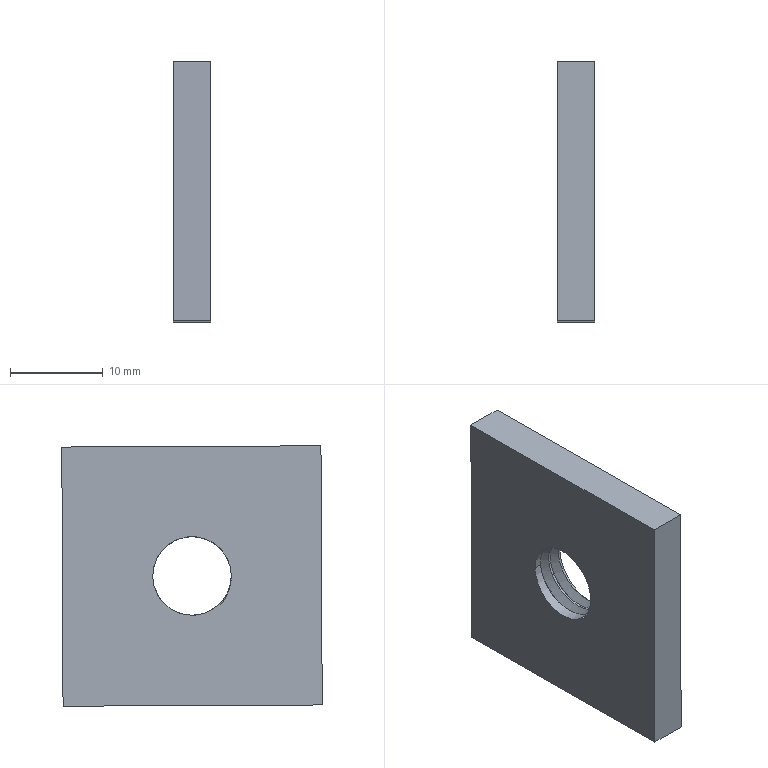Component | SolidWorks | GroundingDeviceAssembly-1_GroundingCopperBlock-1 | 1 solid | 16 faces | box 4 x 28.13 x 28.13 mm | volume 2875 mm3 | cylinder 7 | plane 7 | spline 2 | commonest cylinder face diameters 8.5 x7
STEP:
#1=COLOUR_RGB('',0.7922,0.8196,0.9333);
#2=FILL_AREA_STYLE_COLOUR('',#1);
#3=FILL_AREA_STYLE('',(#2));
#4=SURFACE_STYLE_FILL_AREA(#3);
#5=SURFACE_SIDE_STYLE('',(#4));
#6=SURFACE_STYLE_USAGE(.BOTH.,#5);
#7=PRESENTATION_STYLE_ASSIGNMENT((#6));
#8=CARTESIAN_POINT('',(29.241,-7.002,9.527));
#9=VERTEX_POINT('',#8);
#10=CARTESIAN_POINT('',(29.212,-7.337,9.528));
#11=VERTEX_POINT('',#10);
#12=CARTESIAN_POINT('',(29.241,-7.002,9.527));
#13=CARTESIAN_POINT('',(29.238,-7.002,9.596));
#14=CARTESIAN_POINT('',(29.234,-7.051,9.645));
#15=CARTESIAN_POINT('',(29.23,-7.099,9.695));
#16=CARTESIAN_POINT('',(29.227,-7.169,9.695));
#17=CARTESIAN_POINT('',(29.223,-7.238,9.695));
#18=CARTESIAN_POINT('',(29.219,-7.287,9.646));
#19=CARTESIAN_POINT('',(29.216,-7.336,9.598));
#20=CARTESIAN_POINT('',(29.212,-7.337,9.528));
#21=(BOUNDED_CURVE()B_SPLINE_CURVE(2,(#12,#13,#14,#15,#16,#17,#18,#19,#20),.UNSPECIFIED.,.F.,.F.)B_SPLINE_CURVE_WITH_KNOTS((3,2,2,2,3),(0.4583,0.5,0.5417,0.5833,0.625),.UNSPECIFIED.)CURVE()GEOMETRIC_REPRESENTATION_ITEM()RATIONAL_B_SPLINE_CURVE((1.,0.9239,1.,0.9239,1.,0.9239,1.,0.9239,1.))REPRESENTATION_ITEM(''));
#22=EDGE_CURVE('',#9,#11,#21,.T.);
#23=ORIENTED_EDGE('',*,*,#22,.F.);
#24=CARTESIAN_POINT('',(29.251,-7.002,9.527));
#25=VERTEX_POINT('',#24);
#26=CARTESIAN_POINT('',(29.061,-7.002,9.527));
#27=DIRECTION('',(1.,0.,-0.));
#28=VECTOR('',#27,39.37);
#29=LINE('',#26,#28);
#30=EDGE_CURVE('',#9,#25,#29,.T.);
#31=ORIENTED_EDGE('',*,*,#30,.T.);
#32=CARTESIAN_POINT('',(29.222,-7.337,9.528));
#33=VERTEX_POINT('',#32);
#34=CARTESIAN_POINT('',(29.222,-7.337,9.528));
#35=CARTESIAN_POINT('',(29.225,-7.336,9.598));
#36=CARTESIAN_POINT('',(29.229,-7.287,9.646));
#37=CARTESIAN_POINT('',(29.233,-7.238,9.695));
#38=CARTESIAN_POINT('',(29.236,-7.169,9.695));
#39=CARTESIAN_POINT('',(29.24,-7.099,9.695));
#40=CARTESIAN_POINT('',(29.244,-7.051,9.645));
#41=CARTESIAN_POINT('',(29.247,-7.002,9.596));
#42=CARTESIAN_POINT('',(29.251,-7.002,9.527));
#43=(BOUNDED_CURVE()B_SPLINE_CURVE(2,(#34,#35,#36,#37,#38,#39,#40,#41,#42),.UNSPECIFIED.,.F.,.F.)B_SPLINE_CURVE_WITH_KNOTS((3,2,2,2,3),(0.7083,0.75,0.7917,0.8333,0.875),.UNSPECIFIED.)CURVE()GEOMETRIC_REPRESENTATION_ITEM()RATIONAL_B_SPLINE_CURVE((1.,0.9239,1.,0.9239,1.,0.9239,1.,0.9239,1.))REPRESENTATION_ITEM(''));
#44=EDGE_CURVE('',#33,#25,#43,.T.);
#45=ORIENTED_EDGE('',*,*,#44,.F.);
#46=CARTESIAN_POINT('',(29.061,-7.337,9.528));
#47=DIRECTION('',(1.,0.,-0.));
#48=VECTOR('',#47,39.37);
#49=LINE('',#46,#48);
#50=EDGE_CURVE('',#11,#33,#49,.T.);
#51=ORIENTED_EDGE('',*,*,#50,.F.);
#52=EDGE_LOOP('',(#23,#31,#45,#51));
#53=FACE_OUTER_BOUND('',#52,.T.);
#54=CARTESIAN_POINT('',(29.061,-7.169,9.528));
#55=DIRECTION('',(1.,0.,-0.));
#56=DIRECTION('',(0.,-1.,0.004786));
#57=AXIS2_PLACEMENT_3D('',#54,#55,#56);
#58=CYLINDRICAL_SURFACE('',#57,0.1673);
#59=ADVANCED_FACE('',(#53),#58,.F.);
#60=CARTESIAN_POINT('',(29.1,-7.002,9.527));
#61=VERTEX_POINT('',#60);
#62=CARTESIAN_POINT('',(29.1,-7.337,9.528));
#63=VERTEX_POINT('',#62);
#64=CARTESIAN_POINT('',(29.1,-7.169,9.528));
#65=DIRECTION('',(1.,0.,-0.));
#66=DIRECTION('',(0.,-1.,0.004786));
#67=AXIS2_PLACEMENT_3D('',#64,#65,#66);
#68=CIRCLE('',#67,0.1673);
#69=EDGE_CURVE('',#61,#63,#68,.T.);
#70=ORIENTED_EDGE('',*,*,#69,.F.);
#71=CARTESIAN_POINT('',(29.133,-7.002,9.527));
#72=VERTEX_POINT('',#71);
#73=CARTESIAN_POINT('',(29.061,-7.002,9.527));
#74=DIRECTION('',(1.,0.,-0.));
#75=VECTOR('',#74,39.37);
#76=LINE('',#73,#75);
#77=EDGE_CURVE('',#61,#72,#76,.T.);
#78=ORIENTED_EDGE('',*,*,#77,.T.);
#79=CARTESIAN_POINT('',(29.103,-7.337,9.528));
#80=VERTEX_POINT('',#79);
#81=CARTESIAN_POINT('',(29.103,-7.337,9.528));
#82=CARTESIAN_POINT('',(29.107,-7.336,9.598));
#83=CARTESIAN_POINT('',(29.111,-7.287,9.646));
#84=CARTESIAN_POINT('',(29.115,-7.238,9.695));
#85=CARTESIAN_POINT('',(29.118,-7.169,9.695));
#86=CARTESIAN_POINT('',(29.122,-7.099,9.695));
#87=CARTESIAN_POINT('',(29.126,-7.051,9.645));
#88=CARTESIAN_POINT('',(29.129,-7.002,9.596));
#89=CARTESIAN_POINT('',(29.133,-7.002,9.527));
#90=(BOUNDED_CURVE()B_SPLINE_CURVE(2,(#81,#82,#83,#84,#85,#86,#87,#88,#89),.UNSPECIFIED.,.F.,.F.)B_SPLINE_CURVE_WITH_KNOTS((3,2,2,2,3),(0.04167,0.08333,0.125,0.1667,0.2083),.UNSPECIFIED.)CURVE()GEOMETRIC_REPRESENTATION_ITEM()RATIONAL_B_SPLINE_CURVE((1.,0.9239,1.,0.9239,1.,0.9239,1.,0.9239,1.))REPRESENTATION_ITEM(''));
#91=EDGE_CURVE('',#80,#72,#90,.T.);
#92=ORIENTED_EDGE('',*,*,#91,.F.);
#93=CARTESIAN_POINT('',(29.061,-7.337,9.528));
#94=DIRECTION('',(1.,0.,-0.));
#95=VECTOR('',#94,39.37);
#96=LINE('',#93,#95);
#97=EDGE_CURVE('',#63,#80,#96,.T.);
#98=ORIENTED_EDGE('',*,*,#97,.F.);
#99=EDGE_LOOP('',(#70,#78,#92,#98));
#100=FACE_OUTER_BOUND('',#99,.T.);
#101=CARTESIAN_POINT('',(29.061,-7.169,9.528));
#102=DIRECTION('',(1.,0.,-0.));
#103=DIRECTION('',(0.,-1.,0.004786));
#104=AXIS2_PLACEMENT_3D('',#101,#102,#103);
#105=CYLINDRICAL_SURFACE('',#104,0.1673);
#106=ADVANCED_FACE('',(#100),#105,.F.);
#107=CARTESIAN_POINT('',(29.182,-7.002,9.527));
#108=VERTEX_POINT('',#107);
#109=CARTESIAN_POINT('',(29.153,-7.337,9.528));
#110=VERTEX_POINT('',#109);
#111=CARTESIAN_POINT('',(29.182,-7.002,9.527));
#112=CARTESIAN_POINT('',(29.179,-7.002,9.596));
#113=CARTESIAN_POINT('',(29.175,-7.051,9.645));
#114=CARTESIAN_POINT('',(29.171,-7.099,9.695));
#115=CARTESIAN_POINT('',(29.168,-7.169,9.695));
#116=CARTESIAN_POINT('',(29.164,-7.238,9.695));
#117=CARTESIAN_POINT('',(29.16,-7.287,9.646));
#118=CARTESIAN_POINT('',(29.157,-7.336,9.598));
#119=CARTESIAN_POINT('',(29.153,-7.337,9.528));
#120=(BOUNDED_CURVE()B_SPLINE_CURVE(2,(#111,#112,#113,#114,#115,#116,#117,#118,#119),.UNSPECIFIED.,.F.,.F.)B_SPLINE_CURVE_WITH_KNOTS((3,2,2,2,3),(0.7917,0.8333,0.875,0.9167,0.9583),.UNSPECIFIED.)CURVE()GEOMETRIC_REPRESENTATION_ITEM()RATIONAL_B_SPLINE_CURVE((1.,0.9239,1.,0.9239,1.,0.9239,1.,0.9239,1.))REPRESENTATION_ITEM(''));
#121=EDGE_CURVE('',#108,#110,#120,.T.);
#122=ORIENTED_EDGE('',*,*,#121,.F.);
#123=CARTESIAN_POINT('',(29.192,-7.002,9.527));
#124=VERTEX_POINT('',#123);
#125=CARTESIAN_POINT('',(29.061,-7.002,9.527));
#126=DIRECTION('',(1.,0.,-0.));
#127=VECTOR('',#126,39.37);
#128=LINE('',#125,#127);
#129=EDGE_CURVE('',#108,#124,#128,.T.);
#130=ORIENTED_EDGE('',*,*,#129,.T.);
#131=CARTESIAN_POINT('',(29.163,-7.337,9.528));
#132=VERTEX_POINT('',#131);
#133=CARTESIAN_POINT('',(29.163,-7.337,9.528));
#134=CARTESIAN_POINT('',(29.166,-7.336,9.598));
#135=CARTESIAN_POINT('',(29.17,-7.287,9.646));
#136=CARTESIAN_POINT('',(29.174,-7.238,9.695));
#137=CARTESIAN_POINT('',(29.177,-7.169,9.695));
#138=CARTESIAN_POINT('',(29.181,-7.099,9.695));
#139=CARTESIAN_POINT('',(29.185,-7.051,9.645));
#140=CARTESIAN_POINT('',(29.188,-7.002,9.596));
#141=CARTESIAN_POINT('',(29.192,-7.002,9.527));
#142=(BOUNDED_CURVE()B_SPLINE_CURVE(2,(#133,#134,#135,#136,#137,#138,#139,#140,#141),.UNSPECIFIED.,.F.,.F.)B_SPLINE_CURVE_WITH_KNOTS((3,2,2,2,3),(0.375,0.4167,0.4583,0.5,0.5417),.UNSPECIFIED.)CURVE()GEOMETRIC_REPRESENTATION_ITEM()RATIONAL_B_SPLINE_CURVE((1.,0.9239,1.,0.9239,1.,0.9239,1.,0.9239,1.))REPRESENTATION_ITEM(''));
#143=EDGE_CURVE('',#132,#124,#142,.T.);
#144=ORIENTED_EDGE('',*,*,#143,.F.);
#145=CARTESIAN_POINT('',(29.061,-7.337,9.528));
#146=DIRECTION('',(1.,0.,-0.));
#147=VECTOR('',#146,39.37);
#148=LINE('',#145,#147);
#149=EDGE_CURVE('',#110,#132,#148,.T.);
#150=ORIENTED_EDGE('',*,*,#149,.F.);
#151=EDGE_LOOP('',(#122,#130,#144,#150));
#152=FACE_OUTER_BOUND('',#151,.T.);
#153=CARTESIAN_POINT('',(29.061,-7.169,9.528));
#154=DIRECTION('',(1.,0.,-0.));
#155=DIRECTION('',(0.,-1.,0.004786));
#156=AXIS2_PLACEMENT_3D('',#153,#154,#155);
#157=CYLINDRICAL_SURFACE('',#156,0.1673);
#158=ADVANCED_FACE('',(#152),#157,.F.);
#159=CARTESIAN_POINT('',(29.1,-7.329,9.476));
#160=VERTEX_POINT('',#159);
#161=CARTESIAN_POINT('',(29.1,-7.169,9.528));
#162=DIRECTION('',(1.,0.,-0.));
#163=DIRECTION('',(0.,-1.,0.004786));
#164=AXIS2_PLACEMENT_3D('',#161,#162,#163);
#165=CIRCLE('',#164,0.1673);
#166=EDGE_CURVE('',#63,#160,#165,.T.);
#167=ORIENTED_EDGE('',*,*,#166,.F.);
#168=ORIENTED_EDGE('',*,*,#97,.T.);
#169=CARTESIAN_POINT('',(29.1,-7.329,9.476));
#170=CARTESIAN_POINT('',(29.102,-7.337,9.501));
#171=CARTESIAN_POINT('',(29.103,-7.337,9.528));
#172=(BOUNDED_CURVE()B_SPLINE_CURVE(2,(#169,#170,#171),.UNSPECIFIED.,.F.,.F.)B_SPLINE_CURVE_WITH_KNOTS((3,3),(0.02463,0.04167),.UNSPECIFIED.)CURVE()GEOMETRIC_REPRESENTATION_ITEM()RATIONAL_B_SPLINE_CURVE((0.9632,0.9689,1.))REPRESENTATION_ITEM(''));
#173=EDGE_CURVE('',#160,#80,#172,.T.);
#174=ORIENTED_EDGE('',*,*,#173,.F.);
#175=EDGE_LOOP('',(#167,#168,#174));
#176=FACE_OUTER_BOUND('',#175,.T.);
#177=CARTESIAN_POINT('',(29.061,-7.169,9.528));
#178=DIRECTION('',(1.,0.,-0.));
#179=DIRECTION('',(0.,-1.,0.004786));
#180=AXIS2_PLACEMENT_3D('',#177,#178,#179);
#181=CYLINDRICAL_SURFACE('',#180,0.1673);
#182=ADVANCED_FACE('',(#176),#181,.F.);
#183=ORIENTED_EDGE('',*,*,#77,.F.);
#184=CARTESIAN_POINT('',(29.1,-7.288,9.41));
#185=VERTEX_POINT('',#184);
#186=CARTESIAN_POINT('',(29.1,-7.169,9.528));
#187=DIRECTION('',(1.,0.,-0.));
#188=DIRECTION('',(0.,-1.,0.004786));
#189=AXIS2_PLACEMENT_3D('',#186,#187,#188);
#190=CIRCLE('',#189,0.1673);
#191=EDGE_CURVE('',#185,#61,#190,.T.);
#192=ORIENTED_EDGE('',*,*,#191,.F.);
#193=CARTESIAN_POINT('',(29.145,-7.288,9.41));
#194=VERTEX_POINT('',#193);
#195=CARTESIAN_POINT('',(29.061,-7.288,9.41));
#196=DIRECTION('',(1.,0.,-0.));
#197=VECTOR('',#196,39.37);
#198=LINE('',#195,#197);
#199=EDGE_CURVE('',#185,#194,#198,.T.);
#200=ORIENTED_EDGE('',*,*,#199,.T.);
#201=CARTESIAN_POINT('',(29.153,-7.337,9.528));
#202=CARTESIAN_POINT('',(29.149,-7.337,9.459));
#203=CARTESIAN_POINT('',(29.145,-7.288,9.41));
#204=(BOUNDED_CURVE()B_SPLINE_CURVE(2,(#201,#202,#203),.UNSPECIFIED.,.F.,.F.)B_SPLINE_CURVE_WITH_KNOTS((3,3),(0.9583,1.),.UNSPECIFIED.)CURVE()GEOMETRIC_REPRESENTATION_ITEM()RATIONAL_B_SPLINE_CURVE((1.,0.9239,1.))REPRESENTATION_ITEM(''));
#205=EDGE_CURVE('',#110,#194,#204,.T.);
#206=ORIENTED_EDGE('',*,*,#205,.F.);
#207=ORIENTED_EDGE('',*,*,#149,.T.);
#208=CARTESIAN_POINT('',(29.133,-7.002,9.527));
#209=CARTESIAN_POINT('',(29.137,-7.002,9.457));
#210=CARTESIAN_POINT('',(29.14,-7.052,9.409));
#211=CARTESIAN_POINT('',(29.144,-7.101,9.36));
#212=CARTESIAN_POINT('',(29.148,-7.17,9.36));
#213=CARTESIAN_POINT('',(29.151,-7.24,9.361));
#214=CARTESIAN_POINT('',(29.155,-7.288,9.41));
#215=CARTESIAN_POINT('',(29.159,-7.337,9.459));
#216=CARTESIAN_POINT('',(29.163,-7.337,9.528));
#217=(BOUNDED_CURVE()B_SPLINE_CURVE(2,(#208,#209,#210,#211,#212,#213,#214,#215,#216),.UNSPECIFIED.,.F.,.F.)B_SPLINE_CURVE_WITH_KNOTS((3,2,2,2,3),(0.2083,0.25,0.2917,0.3333,0.375),.UNSPECIFIED.)CURVE()GEOMETRIC_REPRESENTATION_ITEM()RATIONAL_B_SPLINE_CURVE((1.,0.9239,1.,0.9239,1.,0.9239,1.,0.9239,1.))REPRESENTATION_ITEM(''));
#218=EDGE_CURVE('',#72,#132,#217,.T.);
#219=ORIENTED_EDGE('',*,*,#218,.F.);
#220=EDGE_LOOP('',(#183,#192,#200,#206,#207,#219));
#221=FACE_OUTER_BOUND('',#220,.T.);
#222=CARTESIAN_POINT('',(29.061,-7.169,9.528));
#223=DIRECTION('',(1.,0.,-0.));
#224=DIRECTION('',(0.,-1.,0.004786));
#225=AXIS2_PLACEMENT_3D('',#222,#223,#224);
#226=CYLINDRICAL_SURFACE('',#225,0.1673);
#227=ADVANCED_FACE('',(#221),#226,.F.);
#228=ORIENTED_EDGE('',*,*,#129,.F.);
#229=CARTESIAN_POINT('',(29.212,-7.337,9.528));
#230=CARTESIAN_POINT('',(29.208,-7.337,9.459));
#231=CARTESIAN_POINT('',(29.205,-7.288,9.41));
#232=CARTESIAN_POINT('',(29.201,-7.24,9.361));
#233=CARTESIAN_POINT('',(29.197,-7.17,9.36));
#234=CARTESIAN_POINT('',(29.193,-7.101,9.36));
#235=CARTESIAN_POINT('',(29.19,-7.052,9.409));
#236=CARTESIAN_POINT('',(29.186,-7.002,9.457));
#237=CARTESIAN_POINT('',(29.182,-7.002,9.527));
#238=(BOUNDED_CURVE()B_SPLINE_CURVE(2,(#229,#230,#231,#232,#233,#234,#235,#236,#237),.UNSPECIFIED.,.F.,.F.)B_SPLINE_CURVE_WITH_KNOTS((3,2,2,2,3),(0.625,0.6667,0.7083,0.75,0.7917),.UNSPECIFIED.)CURVE()GEOMETRIC_REPRESENTATION_ITEM()RATIONAL_B_SPLINE_CURVE((1.,0.9239,1.,0.9239,1.,0.9239,1.,0.9239,1.))REPRESENTATION_ITEM(''));
#239=EDGE_CURVE('',#11,#108,#238,.T.);
#240=ORIENTED_EDGE('',*,*,#239,.F.);
#241=ORIENTED_EDGE('',*,*,#50,.T.);
#242=CARTESIAN_POINT('',(29.192,-7.002,9.527));
#243=CARTESIAN_POINT('',(29.196,-7.002,9.457));
#244=CARTESIAN_POINT('',(29.199,-7.052,9.409));
#245=CARTESIAN_POINT('',(29.203,-7.101,9.36));
#246=CARTESIAN_POINT('',(29.207,-7.17,9.36));
#247=CARTESIAN_POINT('',(29.211,-7.24,9.361));
#248=CARTESIAN_POINT('',(29.214,-7.288,9.41));
#249=CARTESIAN_POINT('',(29.218,-7.337,9.459));
#250=CARTESIAN_POINT('',(29.222,-7.337,9.528));
#251=(BOUNDED_CURVE()B_SPLINE_CURVE(2,(#242,#243,#244,#245,#246,#247,#248,#249,#250),.UNSPECIFIED.,.F.,.F.)B_SPLINE_CURVE_WITH_KNOTS((3,2,2,2,3),(0.5417,0.5833,0.625,0.6667,0.7083),.UNSPECIFIED.)CURVE()GEOMETRIC_REPRESENTATION_ITEM()RATIONAL_B_SPLINE_CURVE((1.,0.9239,1.,0.9239,1.,0.9239,1.,0.9239,1.))REPRESENTATION_ITEM(''));
#252=EDGE_CURVE('',#124,#33,#251,.T.);
#253=ORIENTED_EDGE('',*,*,#252,.F.);
#254=EDGE_LOOP('',(#228,#240,#241,#253));
#255=FACE_OUTER_BOUND('',#254,.T.);
#256=CARTESIAN_POINT('',(29.061,-7.169,9.528));
#257=DIRECTION('',(1.,0.,-0.));
#258=DIRECTION('',(0.,-1.,0.004786));
#259=AXIS2_PLACEMENT_3D('',#256,#257,#258);
#260=CYLINDRICAL_SURFACE('',#259,0.1673);
#261=ADVANCED_FACE('',(#255),#260,.F.);
#262=CARTESIAN_POINT('',(29.1,-7.723,8.979));
#263=VERTEX_POINT('',#262);
#264=CARTESIAN_POINT('',(29.258,-7.723,8.979));
#265=VERTEX_POINT('',#264);
#266=CARTESIAN_POINT('',(29.1,-7.723,8.979));
#267=DIRECTION('',(1.,0.,-0.));
#268=VECTOR('',#267,39.37);
#269=LINE('',#266,#268);
#270=EDGE_CURVE('',#263,#265,#269,.T.);
#271=ORIENTED_EDGE('',*,*,#270,.T.);
#272=CARTESIAN_POINT('',(29.258,-7.718,10.081));
#273=VERTEX_POINT('',#272);
#274=CARTESIAN_POINT('',(29.258,-7.723,8.979));
#275=DIRECTION('',(-0.,-0.004786,-1.));
#276=VECTOR('',#275,39.37);
#277=LINE('',#274,#276);
#278=EDGE_CURVE('',#273,#265,#277,.T.);
#279=ORIENTED_EDGE('',*,*,#278,.F.);
#280=CARTESIAN_POINT('',(29.1,-7.718,10.081));
#281=VERTEX_POINT('',#280);
#282=CARTESIAN_POINT('',(29.1,-7.718,10.081));
#283=DIRECTION('',(1.,0.,-0.));
#284=VECTOR('',#283,39.37);
#285=LINE('',#282,#284);
#286=EDGE_CURVE('',#281,#273,#285,.T.);
#287=ORIENTED_EDGE('',*,*,#286,.F.);
#288=CARTESIAN_POINT('',(29.1,-7.723,8.979));
#289=DIRECTION('',(-0.,-0.004786,-1.));
#290=VECTOR('',#289,39.37);
#291=LINE('',#288,#290);
#292=EDGE_CURVE('',#281,#263,#291,.T.);
#293=ORIENTED_EDGE('',*,*,#292,.T.);
#294=EDGE_LOOP('',(#271,#279,#287,#293));
#295=FACE_OUTER_BOUND('',#294,.T.);
#296=CARTESIAN_POINT('',(29.1,-7.723,8.979));
#297=DIRECTION('',(0.,-1.,0.004786));
#298=DIRECTION('',(-0.,-0.004786,-1.));
#299=AXIS2_PLACEMENT_3D('',#296,#297,#298);
#300=PLANE('',#299);
#301=ADVANCED_FACE('',(#295),#300,.T.);
#302=ORIENTED_EDGE('',*,*,#286,.T.);
#303=CARTESIAN_POINT('',(29.258,-6.616,10.076));
#304=VERTEX_POINT('',#303);
#305=CARTESIAN_POINT('',(29.258,-6.616,10.076));
#306=DIRECTION('',(0.,-1.,0.004786));
#307=VECTOR('',#306,39.37);
#308=LINE('',#305,#307);
#309=EDGE_CURVE('',#304,#273,#308,.T.);
#310=ORIENTED_EDGE('',*,*,#309,.F.);
#311=CARTESIAN_POINT('',(29.1,-6.616,10.076));
#312=VERTEX_POINT('',#311);
#313=CARTESIAN_POINT('',(29.1,-6.616,10.076));
#314=DIRECTION('',(1.,0.,-0.));
#315=VECTOR('',#314,39.37);
#316=LINE('',#313,#315);
#317=EDGE_CURVE('',#312,#304,#316,.T.);
#318=ORIENTED_EDGE('',*,*,#317,.F.);
#319=CARTESIAN_POINT('',(29.1,-6.616,10.076));
#320=DIRECTION('',(0.,-1.,0.004786));
#321=VECTOR('',#320,39.37);
#322=LINE('',#319,#321);
#323=EDGE_CURVE('',#312,#281,#322,.T.);
#324=ORIENTED_EDGE('',*,*,#323,.T.);
#325=EDGE_LOOP('',(#302,#310,#318,#324));
#326=FACE_OUTER_BOUND('',#325,.T.);
#327=CARTESIAN_POINT('',(29.1,-6.616,10.076));
#328=DIRECTION('',(0.,0.004786,1.));
#329=DIRECTION('',(-1.,-0.,0.));
#330=AXIS2_PLACEMENT_3D('',#327,#328,#329);
#331=PLANE('',#330);
#332=ADVANCED_FACE('',(#326),#331,.T.);
#333=ORIENTED_EDGE('',*,*,#317,.T.);
#334=CARTESIAN_POINT('',(29.258,-6.621,8.974));
#335=VERTEX_POINT('',#334);
#336=CARTESIAN_POINT('',(29.258,-6.621,8.974));
#337=DIRECTION('',(0.,0.004786,1.));
#338=VECTOR('',#337,39.37);
#339=LINE('',#336,#338);
#340=EDGE_CURVE('',#335,#304,#339,.T.);
#341=ORIENTED_EDGE('',*,*,#340,.F.);
#342=CARTESIAN_POINT('',(29.1,-6.621,8.974));
#343=VERTEX_POINT('',#342);
#344=CARTESIAN_POINT('',(29.1,-6.621,8.974));
#345=DIRECTION('',(1.,0.,-0.));
#346=VECTOR('',#345,39.37);
#347=LINE('',#344,#346);
#348=EDGE_CURVE('',#343,#335,#347,.T.);
#349=ORIENTED_EDGE('',*,*,#348,.F.);
#350=CARTESIAN_POINT('',(29.1,-6.621,8.974));
#351=DIRECTION('',(0.,0.004786,1.));
#352=VECTOR('',#351,39.37);
#353=LINE('',#350,#352);
#354=EDGE_CURVE('',#343,#312,#353,.T.);
#355=ORIENTED_EDGE('',*,*,#354,.T.);
#356=EDGE_LOOP('',(#333,#341,#349,#355));
#357=FACE_OUTER_BOUND('',#356,.T.);
#358=CARTESIAN_POINT('',(29.1,-6.621,8.974));
#359=DIRECTION('',(-0.,1.,-0.004786));
#360=DIRECTION('',(0.,0.004786,1.));
#361=AXIS2_PLACEMENT_3D('',#358,#359,#360);
#362=PLANE('',#361);
#363=ADVANCED_FACE('',(#357),#362,.T.);
#364=ORIENTED_EDGE('',*,*,#348,.T.);
#365=CARTESIAN_POINT('',(29.258,-6.621,8.974));
#366=DIRECTION('',(-0.,1.,-0.004786));
#367=VECTOR('',#366,39.37);
#368=LINE('',#365,#367);
#369=EDGE_CURVE('',#265,#335,#368,.T.);
#370=ORIENTED_EDGE('',*,*,#369,.F.);
#371=ORIENTED_EDGE('',*,*,#270,.F.);
#372=CARTESIAN_POINT('',(29.1,-6.621,8.974));
#373=DIRECTION('',(-0.,1.,-0.004786));
#374=VECTOR('',#373,39.37);
#375=LINE('',#372,#374);
#376=EDGE_CURVE('',#263,#343,#375,.T.);
#377=ORIENTED_EDGE('',*,*,#376,.T.);
#378=EDGE_LOOP('',(#364,#370,#371,#377));
#379=FACE_OUTER_BOUND('',#378,.T.);
#380=CARTESIAN_POINT('',(29.1,-6.621,8.974));
#381=DIRECTION('',(-0.,-0.004786,-1.));
#382=DIRECTION('',(1.,0.,-0.));
#383=AXIS2_PLACEMENT_3D('',#380,#381,#382);
#384=PLANE('',#383);
#385=ADVANCED_FACE('',(#379),#384,.T.);
#386=CARTESIAN_POINT('',(29.1,-7.292,9.406));
#387=VERTEX_POINT('',#386);
#388=CARTESIAN_POINT('',(29.1,-7.329,9.476));
#389=CARTESIAN_POINT('',(29.1,-7.325,9.463));
#390=CARTESIAN_POINT('',(29.1,-7.321,9.45));
#391=CARTESIAN_POINT('',(29.1,-7.309,9.427));
#392=CARTESIAN_POINT('',(29.1,-7.301,9.416));
#393=CARTESIAN_POINT('',(29.1,-7.292,9.406));
#394=B_SPLINE_CURVE_WITH_KNOTS('',3,(#388,#389,#390,#391,#392,#393),.UNSPECIFIED.,.F.,.F.,(4,2,4),(0.002169,0.003174,0.004179),.UNSPECIFIED.);
#395=EDGE_CURVE('',#160,#387,#394,.T.);
#396=ORIENTED_EDGE('',*,*,#395,.T.);
#397=CARTESIAN_POINT('',(29.1,-7.169,9.528));
#398=DIRECTION('',(0.,0.7105,0.7037));
#399=VECTOR('',#398,39.37);
#400=LINE('',#397,#399);
#401=EDGE_CURVE('',#387,#185,#400,.T.);
#402=ORIENTED_EDGE('',*,*,#401,.T.);
#403=ORIENTED_EDGE('',*,*,#191,.T.);
#404=ORIENTED_EDGE('',*,*,#69,.T.);
#405=ORIENTED_EDGE('',*,*,#166,.T.);
#406=EDGE_LOOP('',(#396,#402,#403,#404,#405));
#407=FACE_BOUND('',#406,.T.);
#408=ORIENTED_EDGE('',*,*,#292,.F.);
#409=ORIENTED_EDGE('',*,*,#323,.F.);
#410=ORIENTED_EDGE('',*,*,#354,.F.);
#411=ORIENTED_EDGE('',*,*,#376,.F.);
#412=EDGE_LOOP('',(#408,#409,#410,#411));
#413=FACE_OUTER_BOUND('',#412,.T.);
#414=CARTESIAN_POINT('',(29.1,-7.718,10.081));
#415=DIRECTION('',(1.,0.,-0.));
#416=DIRECTION('',(0.,-1.,0.004786));
#417=AXIS2_PLACEMENT_3D('',#414,#415,#416);
#418=PLANE('',#417);
#419=ADVANCED_FACE('',(#407,#413),#418,.F.);
#420=CARTESIAN_POINT('',(29.258,-7.233,9.717));
#421=VERTEX_POINT('',#420);
#422=CARTESIAN_POINT('',(29.258,-7.202,9.363));
#423=VERTEX_POINT('',#422);
#424=CARTESIAN_POINT('',(29.258,-7.233,9.717));
#425=CARTESIAN_POINT('',(29.258,-7.252,9.709));
#426=CARTESIAN_POINT('',(29.258,-7.269,9.699));
#427=CARTESIAN_POINT('',(29.258,-7.292,9.68));
#428=CARTESIAN_POINT('',(29.258,-7.299,9.673));
#429=CARTESIAN_POINT('',(29.258,-7.313,9.658));
#430=CARTESIAN_POINT('',(29.258,-7.319,9.65));
#431=CARTESIAN_POINT('',(29.258,-7.33,9.633));
#432=CARTESIAN_POINT('',(29.258,-7.334,9.624));
#433=CARTESIAN_POINT('',(29.258,-7.342,9.605));
#434=CARTESIAN_POINT('',(29.258,-7.346,9.596));
#435=CARTESIAN_POINT('',(29.258,-7.351,9.577));
#436=CARTESIAN_POINT('',(29.258,-7.352,9.567));
#437=CARTESIAN_POINT('',(29.258,-7.354,9.547));
#438=CARTESIAN_POINT('',(29.258,-7.354,9.537));
#439=CARTESIAN_POINT('',(29.258,-7.353,9.517));
#440=CARTESIAN_POINT('',(29.258,-7.351,9.507));
#441=CARTESIAN_POINT('',(29.258,-7.347,9.487));
#442=CARTESIAN_POINT('',(29.258,-7.343,9.477));
#443=CARTESIAN_POINT('',(29.258,-7.336,9.459));
#444=CARTESIAN_POINT('',(29.258,-7.331,9.45));
#445=CARTESIAN_POINT('',(29.258,-7.32,9.433));
#446=CARTESIAN_POINT('',(29.258,-7.314,9.425));
#447=CARTESIAN_POINT('',(29.258,-7.3,9.411));
#448=CARTESIAN_POINT('',(29.258,-7.293,9.404));
#449=CARTESIAN_POINT('',(29.258,-7.277,9.391));
#450=CARTESIAN_POINT('',(29.258,-7.268,9.386));
#451=CARTESIAN_POINT('',(29.258,-7.251,9.377));
#452=CARTESIAN_POINT('',(29.258,-7.241,9.373));
#453=CARTESIAN_POINT('',(29.258,-7.222,9.367));
#454=CARTESIAN_POINT('',(29.258,-7.212,9.365));
#455=CARTESIAN_POINT('',(29.258,-7.202,9.363));
#456=B_SPLINE_CURVE_WITH_KNOTS('',3,(#424,#425,#426,#427,#428,#429,#430,#431,#432,#433,#434,#435,#436,#437,#438,#439,#440,#441,#442,#443,#444,#445,#446,#447,#448,#449,#450,#451,#452,#453,#454,#455),.UNSPECIFIED.,.F.,.F.,(4,2,2,2,2,2,2,2,2,2,2,2,2,2,2,4),(0.,0.001522,0.002283,0.003043,0.003804,0.004565,0.005326,0.006087,0.006848,0.007608,0.008369,0.00913,0.009891,0.01065,0.01141,0.01217),.UNSPECIFIED.);
#457=EDGE_CURVE('',#421,#423,#456,.T.);
#458=ORIENTED_EDGE('',*,*,#457,.F.);
#459=CARTESIAN_POINT('',(29.258,-7.045,9.416));
#460=VERTEX_POINT('',#459);
#461=CARTESIAN_POINT('',(29.258,-7.045,9.416));
#462=CARTESIAN_POINT('',(29.258,-7.038,9.423));
#463=CARTESIAN_POINT('',(29.258,-7.031,9.43));
#464=CARTESIAN_POINT('',(29.258,-7.019,9.447));
#465=CARTESIAN_POINT('',(29.258,-7.014,9.455));
#466=CARTESIAN_POINT('',(29.258,-7.005,9.473));
#467=CARTESIAN_POINT('',(29.258,-7.002,9.483));
#468=CARTESIAN_POINT('',(29.258,-6.996,9.502));
#469=CARTESIAN_POINT('',(29.258,-6.995,9.512));
#470=CARTESIAN_POINT('',(29.258,-6.993,9.532));
#471=CARTESIAN_POINT('',(29.258,-6.993,9.542));
#472=CARTESIAN_POINT('',(29.258,-6.994,9.562));
#473=CARTESIAN_POINT('',(29.258,-6.996,9.572));
#474=CARTESIAN_POINT('',(29.258,-7.,9.592));
#475=CARTESIAN_POINT('',(29.258,-7.003,9.602));
#476=CARTESIAN_POINT('',(29.258,-7.011,9.62));
#477=CARTESIAN_POINT('',(29.258,-7.016,9.629));
#478=CARTESIAN_POINT('',(29.258,-7.027,9.646));
#479=CARTESIAN_POINT('',(29.258,-7.033,9.654));
#480=CARTESIAN_POINT('',(29.258,-7.047,9.669));
#481=CARTESIAN_POINT('',(29.258,-7.054,9.675));
#482=CARTESIAN_POINT('',(29.258,-7.07,9.688));
#483=CARTESIAN_POINT('',(29.258,-7.078,9.694));
#484=CARTESIAN_POINT('',(29.258,-7.096,9.704));
#485=CARTESIAN_POINT('',(29.258,-7.105,9.708));
#486=CARTESIAN_POINT('',(29.258,-7.123,9.715));
#487=CARTESIAN_POINT('',(29.258,-7.133,9.718));
#488=CARTESIAN_POINT('',(29.258,-7.153,9.722));
#489=CARTESIAN_POINT('',(29.258,-7.163,9.723));
#490=CARTESIAN_POINT('',(29.258,-7.183,9.724));
#491=CARTESIAN_POINT('',(29.258,-7.193,9.723));
#492=CARTESIAN_POINT('',(29.258,-7.213,9.721));
#493=CARTESIAN_POINT('',(29.258,-7.223,9.719));
#494=CARTESIAN_POINT('',(29.258,-7.233,9.717));
#495=B_SPLINE_CURVE_WITH_KNOTS('',3,(#461,#462,#463,#464,#465,#466,#467,#468,#469,#470,#471,#472,#473,#474,#475,#476,#477,#478,#479,#480,#481,#482,#483,#484,#485,#486,#487,#488,#489,#490,#491,#492,#493,#494),.UNSPECIFIED.,.F.,.F.,(4,2,2,2,2,2,2,2,2,2,2,2,2,2,2,2,4),(0.00215,0.002914,0.003678,0.004442,0.005205,0.005969,0.006733,0.007497,0.008261,0.009025,0.009789,0.01055,0.01132,0.01208,0.01284,0.01361,0.01437),.UNSPECIFIED.);
#496=EDGE_CURVE('',#460,#421,#495,.T.);
#497=ORIENTED_EDGE('',*,*,#496,.F.);
#498=CARTESIAN_POINT('',(29.258,-7.169,9.528));
#499=DIRECTION('',(1.,0.,-0.));
#500=DIRECTION('',(0.,-1.,0.004786));
#501=AXIS2_PLACEMENT_3D('',#498,#499,#500);
#502=CIRCLE('',#501,0.1673);
#503=EDGE_CURVE('',#423,#460,#502,.T.);
#504=ORIENTED_EDGE('',*,*,#503,.F.);
#505=EDGE_LOOP('',(#458,#497,#504));
#506=FACE_BOUND('',#505,.T.);
#507=ORIENTED_EDGE('',*,*,#278,.T.);
#508=ORIENTED_EDGE('',*,*,#369,.T.);
#509=ORIENTED_EDGE('',*,*,#340,.T.);
#510=ORIENTED_EDGE('',*,*,#309,.T.);
#511=EDGE_LOOP('',(#507,#508,#509,#510));
#512=FACE_OUTER_BOUND('',#511,.T.);
#513=CARTESIAN_POINT('',(29.258,-7.718,10.081));
#514=DIRECTION('',(1.,0.,-0.));
#515=DIRECTION('',(0.,-1.,0.004786));
#516=AXIS2_PLACEMENT_3D('',#513,#514,#515);
#517=PLANE('',#516);
#518=ADVANCED_FACE('',(#506,#512),#517,.T.);
#519=ORIENTED_EDGE('',*,*,#30,.F.);
#520=CARTESIAN_POINT('',(29.258,-7.202,9.363));
#521=CARTESIAN_POINT('',(29.257,-7.186,9.36));
#522=CARTESIAN_POINT('',(29.256,-7.17,9.36));
#523=CARTESIAN_POINT('',(29.252,-7.101,9.36));
#524=CARTESIAN_POINT('',(29.249,-7.052,9.409));
#525=CARTESIAN_POINT('',(29.245,-7.002,9.457));
#526=CARTESIAN_POINT('',(29.241,-7.002,9.527));
#527=(BOUNDED_CURVE()B_SPLINE_CURVE(2,(#520,#521,#522,#523,#524,#525,#526),.UNSPECIFIED.,.F.,.F.)B_SPLINE_CURVE_WITH_KNOTS((3,2,2,3),(0.3647,0.375,0.4167,0.4583),.UNSPECIFIED.)CURVE()GEOMETRIC_REPRESENTATION_ITEM()RATIONAL_B_SPLINE_CURVE((0.9716,0.9812,1.,0.9239,1.,0.9239,1.))REPRESENTATION_ITEM(''));
#528=EDGE_CURVE('',#423,#9,#527,.T.);
#529=ORIENTED_EDGE('',*,*,#528,.F.);
#530=ORIENTED_EDGE('',*,*,#503,.T.);
#531=CARTESIAN_POINT('',(29.251,-7.002,9.527));
#532=CARTESIAN_POINT('',(29.254,-7.002,9.463));
#533=CARTESIAN_POINT('',(29.258,-7.045,9.416));
#534=(BOUNDED_CURVE()B_SPLINE_CURVE(2,(#531,#532,#533),.UNSPECIFIED.,.F.,.F.)B_SPLINE_CURVE_WITH_KNOTS((3,3),(0.875,0.9135),.UNSPECIFIED.)CURVE()GEOMETRIC_REPRESENTATION_ITEM()RATIONAL_B_SPLINE_CURVE((1.,0.9297,0.9893))REPRESENTATION_ITEM(''));
#535=EDGE_CURVE('',#25,#460,#534,.T.);
#536=ORIENTED_EDGE('',*,*,#535,.F.);
#537=EDGE_LOOP('',(#519,#529,#530,#536));
#538=FACE_OUTER_BOUND('',#537,.T.);
#539=CARTESIAN_POINT('',(29.061,-7.169,9.528));
#540=DIRECTION('',(1.,0.,-0.));
#541=DIRECTION('',(0.,-1.,0.004786));
#542=AXIS2_PLACEMENT_3D('',#539,#540,#541);
#543=CYLINDRICAL_SURFACE('',#542,0.1673);
#544=ADVANCED_FACE('',(#538),#543,.F.);
#545=CARTESIAN_POINT('',(29.121,-7.311,9.387));
#546=VERTEX_POINT('',#545);
#547=CARTESIAN_POINT('',(29.09,-7.282,9.416));
#548=DIRECTION('',(0.6089,-0.5636,-0.5582));
#549=VECTOR('',#548,39.37);
#550=LINE('',#547,#549);
#551=EDGE_CURVE('',#387,#546,#550,.T.);
#552=ORIENTED_EDGE('',*,*,#551,.T.);
#553=CARTESIAN_POINT('',(29.121,-7.311,9.387));
#554=DIRECTION('',(0.6089,0.5636,0.5582));
#555=VECTOR('',#554,39.37);
#556=LINE('',#553,#555);
#557=EDGE_CURVE('',#546,#194,#556,.T.);
#558=ORIENTED_EDGE('',*,*,#557,.T.);
#559=ORIENTED_EDGE('',*,*,#199,.F.);
#560=ORIENTED_EDGE('',*,*,#401,.F.);
#561=EDGE_LOOP('',(#552,#558,#559,#560));
#562=FACE_OUTER_BOUND('',#561,.T.);
#563=CARTESIAN_POINT('',(29.121,-7.311,9.387));
#564=DIRECTION('',(-0.,0.7037,-0.7105));
#565=DIRECTION('',(1.,0.,-0.));
#566=AXIS2_PLACEMENT_3D('',#563,#564,#565);
#567=PLANE('',#566);
#568=ADVANCED_FACE('',(#562),#567,.F.);
#569=ORIENTED_EDGE('',*,*,#173,.T.);
#570=ORIENTED_EDGE('',*,*,#91,.T.);
#571=ORIENTED_EDGE('',*,*,#218,.T.);
#572=ORIENTED_EDGE('',*,*,#143,.T.);
#573=ORIENTED_EDGE('',*,*,#252,.T.);
#574=ORIENTED_EDGE('',*,*,#44,.T.);
#575=ORIENTED_EDGE('',*,*,#535,.T.);
#576=ORIENTED_EDGE('',*,*,#496,.T.);
#577=CARTESIAN_POINT('',(29.121,-7.311,9.387));
#578=CARTESIAN_POINT('',(29.124,-7.369,9.446));
#579=CARTESIAN_POINT('',(29.128,-7.369,9.529));
#580=CARTESIAN_POINT('',(29.132,-7.369,9.611));
#581=CARTESIAN_POINT('',(29.136,-7.31,9.669));
#582=CARTESIAN_POINT('',(29.139,-7.251,9.727));
#583=CARTESIAN_POINT('',(29.143,-7.169,9.727));
#584=CARTESIAN_POINT('',(29.147,-7.086,9.727));
#585=CARTESIAN_POINT('',(29.15,-7.028,9.668));
#586=CARTESIAN_POINT('',(29.154,-6.97,9.609));
#587=CARTESIAN_POINT('',(29.158,-6.97,9.527));
#588=CARTESIAN_POINT('',(29.161,-6.97,9.444));
#589=CARTESIAN_POINT('',(29.165,-7.029,9.386));
#590=CARTESIAN_POINT('',(29.169,-7.088,9.328));
#591=CARTESIAN_POINT('',(29.172,-7.17,9.328));
#592=CARTESIAN_POINT('',(29.176,-7.253,9.328));
#593=CARTESIAN_POINT('',(29.18,-7.311,9.387));
#594=CARTESIAN_POINT('',(29.184,-7.369,9.446));
#595=CARTESIAN_POINT('',(29.187,-7.369,9.529));
#596=CARTESIAN_POINT('',(29.191,-7.369,9.611));
#597=CARTESIAN_POINT('',(29.195,-7.31,9.669));
#598=CARTESIAN_POINT('',(29.198,-7.251,9.727));
#599=CARTESIAN_POINT('',(29.202,-7.169,9.727));
#600=CARTESIAN_POINT('',(29.206,-7.086,9.727));
#601=CARTESIAN_POINT('',(29.209,-7.028,9.668));
#602=CARTESIAN_POINT('',(29.213,-6.97,9.609));
#603=CARTESIAN_POINT('',(29.217,-6.97,9.527));
#604=CARTESIAN_POINT('',(29.22,-6.97,9.444));
#605=CARTESIAN_POINT('',(29.224,-7.029,9.386));
#606=CARTESIAN_POINT('',(29.228,-7.088,9.328));
#607=CARTESIAN_POINT('',(29.232,-7.17,9.328));
#608=CARTESIAN_POINT('',(29.235,-7.253,9.328));
#609=CARTESIAN_POINT('',(29.239,-7.311,9.387));
#610=CARTESIAN_POINT('',(29.243,-7.369,9.446));
#611=CARTESIAN_POINT('',(29.246,-7.369,9.529));
#612=CARTESIAN_POINT('',(29.25,-7.369,9.611));
#613=CARTESIAN_POINT('',(29.254,-7.31,9.669));
#614=CARTESIAN_POINT('',(29.256,-7.277,9.702));
#615=CARTESIAN_POINT('',(29.258,-7.233,9.717));
#616=(BOUNDED_CURVE()B_SPLINE_CURVE(2,(#577,#578,#579,#580,#581,#582,#583,#584,#585,#586,#587,#588,#589,#590,#591,#592,#593,#594,#595,#596,#597,#598,#599,#600,#601,#602,#603,#604,#605,#606,#607,#608,#609,#610,#611,#612,#613,#614,#615),.UNSPECIFIED.,.F.,.F.)B_SPLINE_CURVE_WITH_KNOTS((3,2,2,2,2,2,2,2,2,2,2,2,2,2,2,2,2,2,2,3),(0.,0.04167,0.08333,0.125,0.1667,0.2083,0.25,0.2917,0.3333,0.375,0.4167,0.4583,0.5,0.5417,0.5833,0.625,0.6667,0.7083,0.75,0.7742),.UNSPECIFIED.)CURVE()GEOMETRIC_REPRESENTATION_ITEM()RATIONAL_B_SPLINE_CURVE((1.,0.9239,1.,0.9239,1.,0.9239,1.,0.9239,1.,0.9239,1.,0.9239,1.,0.9239,1.,0.9239,1.,0.9239,1.,0.9239,1.,0.9239,1.,0.9239,1.,0.9239,1.,0.9239,1.,0.9239,1.,0.9239,1.,0.9239,1.,0.9239,1.,0.9558,0.9629))REPRESENTATION_ITEM(''));
#617=EDGE_CURVE('',#546,#421,#616,.T.);
#618=ORIENTED_EDGE('',*,*,#617,.F.);
#619=ORIENTED_EDGE('',*,*,#551,.F.);
#620=ORIENTED_EDGE('',*,*,#395,.F.);
#621=EDGE_LOOP('',(#569,#570,#571,#572,#573,#574,#575,#576,#618,#619,#620));
#622=FACE_OUTER_BOUND('',#621,.T.);
#623=CARTESIAN_POINT('',(29.091,-7.284,9.414));
#624=CARTESIAN_POINT('',(29.095,-7.331,9.462));
#625=CARTESIAN_POINT('',(29.099,-7.33,9.528));
#626=CARTESIAN_POINT('',(29.102,-7.33,9.595));
#627=CARTESIAN_POINT('',(29.106,-7.283,9.642));
#628=CARTESIAN_POINT('',(29.11,-7.235,9.689));
#629=CARTESIAN_POINT('',(29.113,-7.169,9.689));
#630=CARTESIAN_POINT('',(29.117,-7.102,9.688));
#631=CARTESIAN_POINT('',(29.121,-7.055,9.641));
#632=CARTESIAN_POINT('',(29.124,-7.008,9.593));
#633=CARTESIAN_POINT('',(29.128,-7.008,9.527));
#634=CARTESIAN_POINT('',(29.132,-7.009,9.46));
#635=CARTESIAN_POINT('',(29.136,-7.056,9.413));
#636=CARTESIAN_POINT('',(29.139,-7.104,9.366));
#637=CARTESIAN_POINT('',(29.143,-7.17,9.367));
#638=CARTESIAN_POINT('',(29.147,-7.237,9.367));
#639=CARTESIAN_POINT('',(29.15,-7.284,9.414));
#640=CARTESIAN_POINT('',(29.154,-7.331,9.462));
#641=CARTESIAN_POINT('',(29.158,-7.33,9.528));
#642=CARTESIAN_POINT('',(29.161,-7.33,9.595));
#643=CARTESIAN_POINT('',(29.165,-7.283,9.642));
#644=CARTESIAN_POINT('',(29.169,-7.235,9.689));
#645=CARTESIAN_POINT('',(29.172,-7.169,9.689));
#646=CARTESIAN_POINT('',(29.176,-7.102,9.688));
#647=CARTESIAN_POINT('',(29.18,-7.055,9.641));
#648=CARTESIAN_POINT('',(29.184,-7.008,9.593));
#649=CARTESIAN_POINT('',(29.187,-7.008,9.527));
#650=CARTESIAN_POINT('',(29.191,-7.009,9.46));
#651=CARTESIAN_POINT('',(29.195,-7.056,9.413));
#652=CARTESIAN_POINT('',(29.198,-7.104,9.366));
#653=CARTESIAN_POINT('',(29.202,-7.17,9.367));
#654=CARTESIAN_POINT('',(29.206,-7.237,9.367));
#655=CARTESIAN_POINT('',(29.209,-7.284,9.414));
#656=CARTESIAN_POINT('',(29.213,-7.331,9.462));
#657=CARTESIAN_POINT('',(29.217,-7.33,9.528));
#658=CARTESIAN_POINT('',(29.22,-7.33,9.595));
#659=CARTESIAN_POINT('',(29.224,-7.283,9.642));
#660=CARTESIAN_POINT('',(29.228,-7.235,9.689));
#661=CARTESIAN_POINT('',(29.232,-7.169,9.689));
#662=CARTESIAN_POINT('',(29.235,-7.102,9.688));
#663=CARTESIAN_POINT('',(29.239,-7.055,9.641));
#664=CARTESIAN_POINT('',(29.243,-7.008,9.593));
#665=CARTESIAN_POINT('',(29.246,-7.008,9.527));
#666=CARTESIAN_POINT('',(29.25,-7.009,9.46));
#667=CARTESIAN_POINT('',(29.254,-7.056,9.413));
#668=CARTESIAN_POINT('',(29.257,-7.104,9.366));
#669=CARTESIAN_POINT('',(29.261,-7.17,9.367));
#670=CARTESIAN_POINT('',(29.265,-7.237,9.367));
#671=CARTESIAN_POINT('',(29.268,-7.284,9.414));
#672=CARTESIAN_POINT('',(29.121,-7.311,9.387));
#673=CARTESIAN_POINT('',(29.124,-7.369,9.446));
#674=CARTESIAN_POINT('',(29.128,-7.369,9.529));
#675=CARTESIAN_POINT('',(29.132,-7.369,9.611));
#676=CARTESIAN_POINT('',(29.136,-7.31,9.669));
#677=CARTESIAN_POINT('',(29.139,-7.251,9.727));
#678=CARTESIAN_POINT('',(29.143,-7.169,9.727));
#679=CARTESIAN_POINT('',(29.147,-7.086,9.727));
#680=CARTESIAN_POINT('',(29.15,-7.028,9.668));
#681=CARTESIAN_POINT('',(29.154,-6.97,9.609));
#682=CARTESIAN_POINT('',(29.158,-6.97,9.527));
#683=CARTESIAN_POINT('',(29.161,-6.97,9.444));
#684=CARTESIAN_POINT('',(29.165,-7.029,9.386));
#685=CARTESIAN_POINT('',(29.169,-7.088,9.328));
#686=CARTESIAN_POINT('',(29.172,-7.17,9.328));
#687=CARTESIAN_POINT('',(29.176,-7.253,9.328));
#688=CARTESIAN_POINT('',(29.18,-7.311,9.387));
#689=CARTESIAN_POINT('',(29.184,-7.369,9.446));
#690=CARTESIAN_POINT('',(29.187,-7.369,9.529));
#691=CARTESIAN_POINT('',(29.191,-7.369,9.611));
#692=CARTESIAN_POINT('',(29.195,-7.31,9.669));
#693=CARTESIAN_POINT('',(29.198,-7.251,9.727));
#694=CARTESIAN_POINT('',(29.202,-7.169,9.727));
#695=CARTESIAN_POINT('',(29.206,-7.086,9.727));
#696=CARTESIAN_POINT('',(29.209,-7.028,9.668));
#697=CARTESIAN_POINT('',(29.213,-6.97,9.609));
#698=CARTESIAN_POINT('',(29.217,-6.97,9.527));
#699=CARTESIAN_POINT('',(29.22,-6.97,9.444));
#700=CARTESIAN_POINT('',(29.224,-7.029,9.386));
#701=CARTESIAN_POINT('',(29.228,-7.088,9.328));
#702=CARTESIAN_POINT('',(29.232,-7.17,9.328));
#703=CARTESIAN_POINT('',(29.235,-7.253,9.328));
#704=CARTESIAN_POINT('',(29.239,-7.311,9.387));
#705=CARTESIAN_POINT('',(29.243,-7.369,9.446));
#706=CARTESIAN_POINT('',(29.246,-7.369,9.529));
#707=CARTESIAN_POINT('',(29.25,-7.369,9.611));
#708=CARTESIAN_POINT('',(29.254,-7.31,9.669));
#709=CARTESIAN_POINT('',(29.257,-7.251,9.727));
#710=CARTESIAN_POINT('',(29.261,-7.169,9.727));
#711=CARTESIAN_POINT('',(29.265,-7.086,9.727));
#712=CARTESIAN_POINT('',(29.268,-7.028,9.668));
#713=CARTESIAN_POINT('',(29.272,-6.97,9.609));
#714=CARTESIAN_POINT('',(29.276,-6.97,9.527));
#715=CARTESIAN_POINT('',(29.279,-6.97,9.444));
#716=CARTESIAN_POINT('',(29.283,-7.029,9.386));
#717=CARTESIAN_POINT('',(29.287,-7.088,9.328));
#718=CARTESIAN_POINT('',(29.291,-7.17,9.328));
#719=CARTESIAN_POINT('',(29.294,-7.253,9.328));
#720=CARTESIAN_POINT('',(29.298,-7.311,9.387));
#721=(BOUNDED_SURFACE()B_SPLINE_SURFACE(1,2,((#623,#624,#625,#626,#627,#628,#629,#630,#631,#632,#633,#634,#635,#636,#637,#638,#639,#640,#641,#642,#643,#644,#645,#646,#647,#648,#649,#650,#651,#652,#653,#654,#655,#656,#657,#658,#659,#660,#661,#662,#663,#664,#665,#666,#667,#668,#669,#670,#671),(#672,#673,#674,#675,#676,#677,#678,#679,#680,#681,#682,#683,#684,#685,#686,#687,#688,#689,#690,#691,#692,#693,#694,#695,#696,#697,#698,#699,#700,#701,#702,#703,#704,#705,#706,#707,#708,#709,#710,#711,#712,#713,#714,#715,#716,#717,#718,#719,#720)),.UNSPECIFIED.,.F.,.F.,.F.)B_SPLINE_SURFACE_WITH_KNOTS((2,2),(3,2,2,2,2,2,2,2,2,2,2,2,2,2,2,2,2,2,2,2,2,2,2,2,3),(0.,1.),(0.,0.04167,0.08333,0.125,0.1667,0.2083,0.25,0.2917,0.3333,0.375,0.4167,0.4583,0.5,0.5417,0.5833,0.625,0.6667,0.7083,0.75,0.7917,0.8333,0.875,0.9167,0.9583,1.),.UNSPECIFIED.)GEOMETRIC_REPRESENTATION_ITEM()RATIONAL_B_SPLINE_SURFACE(((1.,0.9239,1.,0.9239,1.,0.9239,1.,0.9239,1.,0.9239,1.,0.9239,1.,0.9239,1.,0.9239,1.,0.9239,1.,0.9239,1.,0.9239,1.,0.9239,1.,0.9239,1.,0.9239,1.,0.9239,1.,0.9239,1.,0.9239,1.,0.9239,1.,0.9239,1.,0.9239,1.,0.9239,1.,0.9239,1.,0.9239,1.,0.9239,1.),(1.,0.9239,1.,0.9239,1.,0.9239,1.,0.9239,1.,0.9239,1.,0.9239,1.,0.9239,1.,0.9239,1.,0.9239,1.,0.9239,1.,0.9239,1.,0.9239,1.,0.9239,1.,0.9239,1.,0.9239,1.,0.9239,1.,0.9239,1.,0.9239,1.,0.9239,1.,0.9239,1.,0.9239,1.,0.9239,1.,0.9239,1.,0.9239,1.)))REPRESENTATION_ITEM('')SURFACE());
#722=ADVANCED_FACE('',(#622),#721,.F.);
#723=ORIENTED_EDGE('',*,*,#457,.T.);
#724=ORIENTED_EDGE('',*,*,#528,.T.);
#725=ORIENTED_EDGE('',*,*,#22,.T.);
#726=ORIENTED_EDGE('',*,*,#239,.T.);
#727=ORIENTED_EDGE('',*,*,#121,.T.);
#728=ORIENTED_EDGE('',*,*,#205,.T.);
#729=ORIENTED_EDGE('',*,*,#557,.F.);
#730=ORIENTED_EDGE('',*,*,#617,.T.);
#731=EDGE_LOOP('',(#723,#724,#725,#726,#727,#728,#729,#730));
#732=FACE_OUTER_BOUND('',#731,.T.);
#733=CARTESIAN_POINT('',(29.121,-7.311,9.387));
#734=CARTESIAN_POINT('',(29.124,-7.369,9.446));
#735=CARTESIAN_POINT('',(29.128,-7.369,9.529));
#736=CARTESIAN_POINT('',(29.132,-7.369,9.611));
#737=CARTESIAN_POINT('',(29.136,-7.31,9.669));
#738=CARTESIAN_POINT('',(29.139,-7.251,9.727));
#739=CARTESIAN_POINT('',(29.143,-7.169,9.727));
#740=CARTESIAN_POINT('',(29.147,-7.086,9.727));
#741=CARTESIAN_POINT('',(29.15,-7.028,9.668));
#742=CARTESIAN_POINT('',(29.154,-6.97,9.609));
#743=CARTESIAN_POINT('',(29.158,-6.97,9.527));
#744=CARTESIAN_POINT('',(29.161,-6.97,9.444));
#745=CARTESIAN_POINT('',(29.165,-7.029,9.386));
#746=CARTESIAN_POINT('',(29.169,-7.088,9.328));
#747=CARTESIAN_POINT('',(29.172,-7.17,9.328));
#748=CARTESIAN_POINT('',(29.176,-7.253,9.328));
#749=CARTESIAN_POINT('',(29.18,-7.311,9.387));
#750=CARTESIAN_POINT('',(29.184,-7.369,9.446));
#751=CARTESIAN_POINT('',(29.187,-7.369,9.529));
#752=CARTESIAN_POINT('',(29.191,-7.369,9.611));
#753=CARTESIAN_POINT('',(29.195,-7.31,9.669));
#754=CARTESIAN_POINT('',(29.198,-7.251,9.727));
#755=CARTESIAN_POINT('',(29.202,-7.169,9.727));
#756=CARTESIAN_POINT('',(29.206,-7.086,9.727));
#757=CARTESIAN_POINT('',(29.209,-7.028,9.668));
#758=CARTESIAN_POINT('',(29.213,-6.97,9.609));
#759=CARTESIAN_POINT('',(29.217,-6.97,9.527));
#760=CARTESIAN_POINT('',(29.22,-6.97,9.444));
#761=CARTESIAN_POINT('',(29.224,-7.029,9.386));
#762=CARTESIAN_POINT('',(29.228,-7.088,9.328));
#763=CARTESIAN_POINT('',(29.232,-7.17,9.328));
#764=CARTESIAN_POINT('',(29.235,-7.253,9.328));
#765=CARTESIAN_POINT('',(29.239,-7.311,9.387));
#766=CARTESIAN_POINT('',(29.243,-7.369,9.446));
#767=CARTESIAN_POINT('',(29.246,-7.369,9.529));
#768=CARTESIAN_POINT('',(29.25,-7.369,9.611));
#769=CARTESIAN_POINT('',(29.254,-7.31,9.669));
#770=CARTESIAN_POINT('',(29.257,-7.251,9.727));
#771=CARTESIAN_POINT('',(29.261,-7.169,9.727));
#772=CARTESIAN_POINT('',(29.265,-7.086,9.727));
#773=CARTESIAN_POINT('',(29.268,-7.028,9.668));
#774=CARTESIAN_POINT('',(29.272,-6.97,9.609));
#775=CARTESIAN_POINT('',(29.276,-6.97,9.527));
#776=CARTESIAN_POINT('',(29.279,-6.97,9.444));
#777=CARTESIAN_POINT('',(29.283,-7.029,9.386));
#778=CARTESIAN_POINT('',(29.287,-7.088,9.328));
#779=CARTESIAN_POINT('',(29.291,-7.17,9.328));
#780=CARTESIAN_POINT('',(29.294,-7.253,9.328));
#781=CARTESIAN_POINT('',(29.298,-7.311,9.387));
#782=CARTESIAN_POINT('',(29.15,-7.284,9.414));
#783=CARTESIAN_POINT('',(29.154,-7.331,9.462));
#784=CARTESIAN_POINT('',(29.158,-7.33,9.528));
#785=CARTESIAN_POINT('',(29.161,-7.33,9.595));
#786=CARTESIAN_POINT('',(29.165,-7.283,9.642));
#787=CARTESIAN_POINT('',(29.169,-7.235,9.689));
#788=CARTESIAN_POINT('',(29.172,-7.169,9.689));
#789=CARTESIAN_POINT('',(29.176,-7.102,9.688));
#790=CARTESIAN_POINT('',(29.18,-7.055,9.641));
#791=CARTESIAN_POINT('',(29.184,-7.008,9.593));
#792=CARTESIAN_POINT('',(29.187,-7.008,9.527));
#793=CARTESIAN_POINT('',(29.191,-7.009,9.46));
#794=CARTESIAN_POINT('',(29.195,-7.056,9.413));
#795=CARTESIAN_POINT('',(29.198,-7.104,9.366));
#796=CARTESIAN_POINT('',(29.202,-7.17,9.367));
#797=CARTESIAN_POINT('',(29.206,-7.237,9.367));
#798=CARTESIAN_POINT('',(29.209,-7.284,9.414));
#799=CARTESIAN_POINT('',(29.213,-7.331,9.462));
#800=CARTESIAN_POINT('',(29.217,-7.33,9.528));
#801=CARTESIAN_POINT('',(29.22,-7.33,9.595));
#802=CARTESIAN_POINT('',(29.224,-7.283,9.642));
#803=CARTESIAN_POINT('',(29.228,-7.235,9.689));
#804=CARTESIAN_POINT('',(29.232,-7.169,9.689));
#805=CARTESIAN_POINT('',(29.235,-7.102,9.688));
#806=CARTESIAN_POINT('',(29.239,-7.055,9.641));
#807=CARTESIAN_POINT('',(29.243,-7.008,9.593));
#808=CARTESIAN_POINT('',(29.246,-7.008,9.527));
#809=CARTESIAN_POINT('',(29.25,-7.009,9.46));
#810=CARTESIAN_POINT('',(29.254,-7.056,9.413));
#811=CARTESIAN_POINT('',(29.257,-7.104,9.366));
#812=CARTESIAN_POINT('',(29.261,-7.17,9.367));
#813=CARTESIAN_POINT('',(29.265,-7.237,9.367));
#814=CARTESIAN_POINT('',(29.268,-7.284,9.414));
#815=CARTESIAN_POINT('',(29.272,-7.331,9.462));
#816=CARTESIAN_POINT('',(29.276,-7.33,9.528));
#817=CARTESIAN_POINT('',(29.279,-7.33,9.595));
#818=CARTESIAN_POINT('',(29.283,-7.283,9.642));
#819=CARTESIAN_POINT('',(29.287,-7.235,9.689));
#820=CARTESIAN_POINT('',(29.291,-7.169,9.689));
#821=CARTESIAN_POINT('',(29.294,-7.102,9.688));
#822=CARTESIAN_POINT('',(29.298,-7.055,9.641));
#823=CARTESIAN_POINT('',(29.302,-7.008,9.593));
#824=CARTESIAN_POINT('',(29.305,-7.008,9.527));
#825=CARTESIAN_POINT('',(29.309,-7.009,9.46));
#826=CARTESIAN_POINT('',(29.313,-7.056,9.413));
#827=CARTESIAN_POINT('',(29.316,-7.104,9.366));
#828=CARTESIAN_POINT('',(29.32,-7.17,9.367));
#829=CARTESIAN_POINT('',(29.324,-7.237,9.367));
#830=CARTESIAN_POINT('',(29.327,-7.284,9.414));
#831=(BOUNDED_SURFACE()B_SPLINE_SURFACE(1,2,((#733,#734,#735,#736,#737,#738,#739,#740,#741,#742,#743,#744,#745,#746,#747,#748,#749,#750,#751,#752,#753,#754,#755,#756,#757,#758,#759,#760,#761,#762,#763,#764,#765,#766,#767,#768,#769,#770,#771,#772,#773,#774,#775,#776,#777,#778,#779,#780,#781),(#782,#783,#784,#785,#786,#787,#788,#789,#790,#791,#792,#793,#794,#795,#796,#797,#798,#799,#800,#801,#802,#803,#804,#805,#806,#807,#808,#809,#810,#811,#812,#813,#814,#815,#816,#817,#818,#819,#820,#821,#822,#823,#824,#825,#826,#827,#828,#829,#830)),.UNSPECIFIED.,.F.,.F.,.F.)B_SPLINE_SURFACE_WITH_KNOTS((2,2),(3,2,2,2,2,2,2,2,2,2,2,2,2,2,2,2,2,2,2,2,2,2,2,2,3),(0.,1.),(0.,0.04167,0.08333,0.125,0.1667,0.2083,0.25,0.2917,0.3333,0.375,0.4167,0.4583,0.5,0.5417,0.5833,0.625,0.6667,0.7083,0.75,0.7917,0.8333,0.875,0.9167,0.9583,1.),.UNSPECIFIED.)GEOMETRIC_REPRESENTATION_ITEM()RATIONAL_B_SPLINE_SURFACE(((1.,0.9239,1.,0.9239,1.,0.9239,1.,0.9239,1.,0.9239,1.,0.9239,1.,0.9239,1.,0.9239,1.,0.9239,1.,0.9239,1.,0.9239,1.,0.9239,1.,0.9239,1.,0.9239,1.,0.9239,1.,0.9239,1.,0.9239,1.,0.9239,1.,0.9239,1.,0.9239,1.,0.9239,1.,0.9239,1.,0.9239,1.,0.9239,1.),(1.,0.9239,1.,0.9239,1.,0.9239,1.,0.9239,1.,0.9239,1.,0.9239,1.,0.9239,1.,0.9239,1.,0.9239,1.,0.9239,1.,0.9239,1.,0.9239,1.,0.9239,1.,0.9239,1.,0.9239,1.,0.9239,1.,0.9239,1.,0.9239,1.,0.9239,1.,0.9239,1.,0.9239,1.,0.9239,1.,0.9239,1.,0.9239,1.)))REPRESENTATION_ITEM('')SURFACE());
#832=ADVANCED_FACE('',(#732),#831,.F.);
#833=CLOSED_SHELL('',(#59,#106,#158,#182,#227,#261,#301,#332,#363,#385,#419,#518,#544,#568,#722,#832));
#834=MANIFOLD_SOLID_BREP('',#833);
#835=STYLED_ITEM('',(#7),#834);
#836=PRESENTATION_LAYER_ASSIGNMENT('','',(#835));
#837=(LENGTH_UNIT()NAMED_UNIT(*)SI_UNIT($,.METRE.));
#838=LENGTH_MEASURE_WITH_UNIT(LENGTH_MEASURE(0.0254),#837);
#839=DIMENSIONAL_EXPONENTS(1.,0.,0.,0.,0.,0.,0.);
#840=(CONVERSION_BASED_UNIT('',#838)LENGTH_UNIT()NAMED_UNIT(#839));
#841=UNCERTAINTY_MEASURE_WITH_UNIT(LENGTH_MEASURE(0.00001),#840,'','');
#842=(NAMED_UNIT(*)PLANE_ANGLE_UNIT()SI_UNIT($,.RADIAN.));
#843=(NAMED_UNIT(*)SI_UNIT($,.STERADIAN.)SOLID_ANGLE_UNIT());
#844=(GEOMETRIC_REPRESENTATION_CONTEXT(3)GLOBAL_UNCERTAINTY_ASSIGNED_CONTEXT((#841))GLOBAL_UNIT_ASSIGNED_CONTEXT((#840,#842,#843))REPRESENTATION_CONTEXT('',''));
#845=MECHANICAL_DESIGN_GEOMETRIC_PRESENTATION_REPRESENTATION('',(#835),#844);
#846=CARTESIAN_POINT('',(0.,0.,0.));
#847=DIRECTION('',(0.,0.,1.));
#848=DIRECTION('',(1.,0.,0.));
#849=AXIS2_PLACEMENT_3D('',#846,#847,#848);
#850=(LENGTH_UNIT()NAMED_UNIT(*)SI_UNIT($,.METRE.));
#851=LENGTH_MEASURE_WITH_UNIT(LENGTH_MEASURE(0.0254),#850);
#852=DIMENSIONAL_EXPONENTS(1.,0.,0.,0.,0.,0.,0.);
#853=(CONVERSION_BASED_UNIT('',#851)LENGTH_UNIT()NAMED_UNIT(#852));
#854=UNCERTAINTY_MEASURE_WITH_UNIT(LENGTH_MEASURE(0.00001),#853,'','');
#855=(NAMED_UNIT(*)PLANE_ANGLE_UNIT()SI_UNIT($,.RADIAN.));
#856=(NAMED_UNIT(*)SI_UNIT($,.STERADIAN.)SOLID_ANGLE_UNIT());
#857=(GEOMETRIC_REPRESENTATION_CONTEXT(3)GLOBAL_UNCERTAINTY_ASSIGNED_CONTEXT((#854))GLOBAL_UNIT_ASSIGNED_CONTEXT((#853,#855,#856))REPRESENTATION_CONTEXT('',''));
#858=ADVANCED_BREP_SHAPE_REPRESENTATION('',(#834,#849),#857);